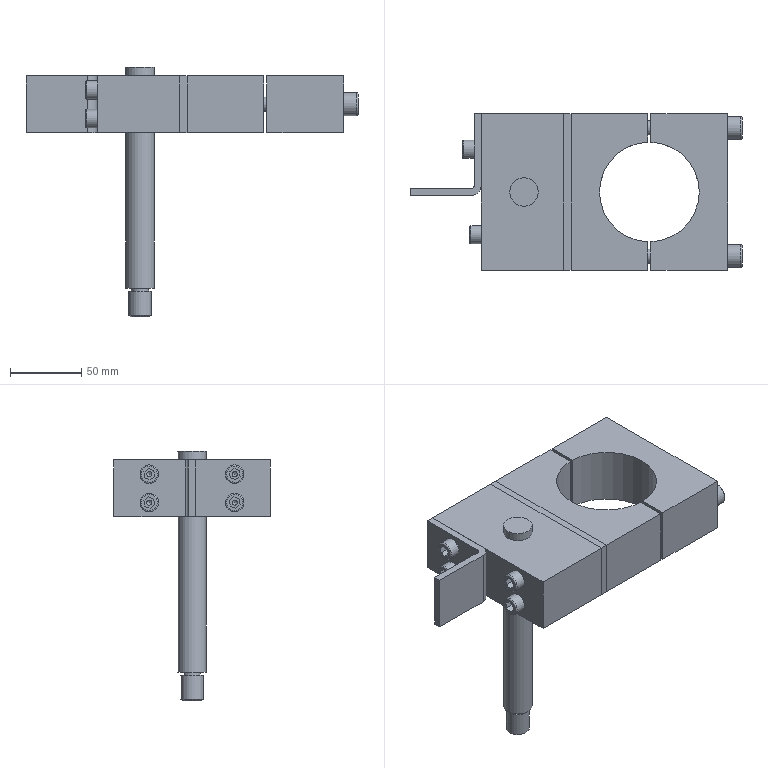Assembly | NX | mm | 12 component files | 12 solids | 181 faces | box 233 x 110 x 175 mm | volume 662385 mm3 | plane 110 | cylinder 40 | cone 25 | torus 6 | commonest cylinder face diameters 9 x10 8 x8 10 x4 13 x4 14 x3 16 x3 20 x2 70 x2
Bill of materials:
CH3404.2-3 | 1 |  | Rectangular block with one larger round hole on the top face and four smaller round holes in a 2x2 pattern on one long side face.
CH3404.2-5 | 1 |  | Thin flat rectangular plate with four round through holes in a 2x2 pattern, two near each end.
CH3404-15 | 1 |  | Stepped solid cylindrical pin: a long main section and a short smaller-diameter end section, with a small neck or groove at the step.
unnamed part 1 | 4 |  | Headed cylindrical pin: a short larger-diameter cylindrical head, a long smooth shank and a chamfered tip.
CH3404.2-2 | 1 |  | Rectangular block with a semicircular cutout running all the way through one long edge, and two round holes through the long side face, one on each side of the cutout.
unnamed part 2 | 2 |  | Cap-screw-like part: a cylindrical head with a hexagonal socket recess, a long smooth cylindrical shank and a chamfered tip.
CH3404.2-4 | 1 |  | L-shaped bent plate bracket of uniform thickness with a rounded inside and outside bend; one leg has two round holes and the other leg has none.
CH3404.2-1 | 1 |  | Rectangular block with a large semicircular cutout open to one long face and running the full height, plus one round hole in each flank beside the cutout; the holes appear to end in cone-shaped bottoms.
Mates:
1. fix | CH3404_2-4 1 component
2. touch align | CH3404_2-3 1 face | CH3404_2-4 1 face
3. touch align | CH3404_2-3 1 | assembly datumplane
4. touch align | CH3404_2-3 1 face | CH3404_2-4 1 face
5. touch align | CH3404_2-1 1 face | CH3404_2-3 1 face
6. distance | CH3404_2-2 1 face | CH3404_2-1 1 face
7. touch align | CH3404_2-2 1 face | CH3404_2-1 1 face
8. touch align | CH3404_2-2 1 face | CH3404_2-1 1 face
9. touch align | GB_T70_1_M10X100 2 face | CH3404_2-2 1 face
10. touch align | GB_T70_1_M10X100 2 face | CH3404_2-2 1 face
11. touch align | GB_T70_1_M10X100 1 face | CH3404_2-2 1 face
12. touch align | GB_T70_1_M10X100 1 face | CH3404_2-2 1 face
13. touch align | CH3404_2-5 1 face | CH3404_2-1 1 face
14. touch align | CH3404_2-5 1 face | CH3404_2-1 1 face
15. touch align | GB_T70_1_M8X80 2 face | CH3404_2-3 1 face
16. touch align | GB_T70_1_M8X80 2 face | CH3404_2-3 1 face
17. touch align | GB_T70_1_M8X80 4 face | CH3404_2-4 1 face
18. touch align | GB_T70_1_M8X80 4 face | CH3404_2-4 1 face
19. touch align | GB_T70_1_M8X80 3 face | CH3404_2-4 1 face
20. touch align | GB_T70_1_M8X80 3 face | CH3404_2-4 1 face
21. touch align | CH3404_2-6 1 face | CH3404_2-3 1 face
22. distance | CH3404_2-6 1 face | CH3404_2-3 1 face